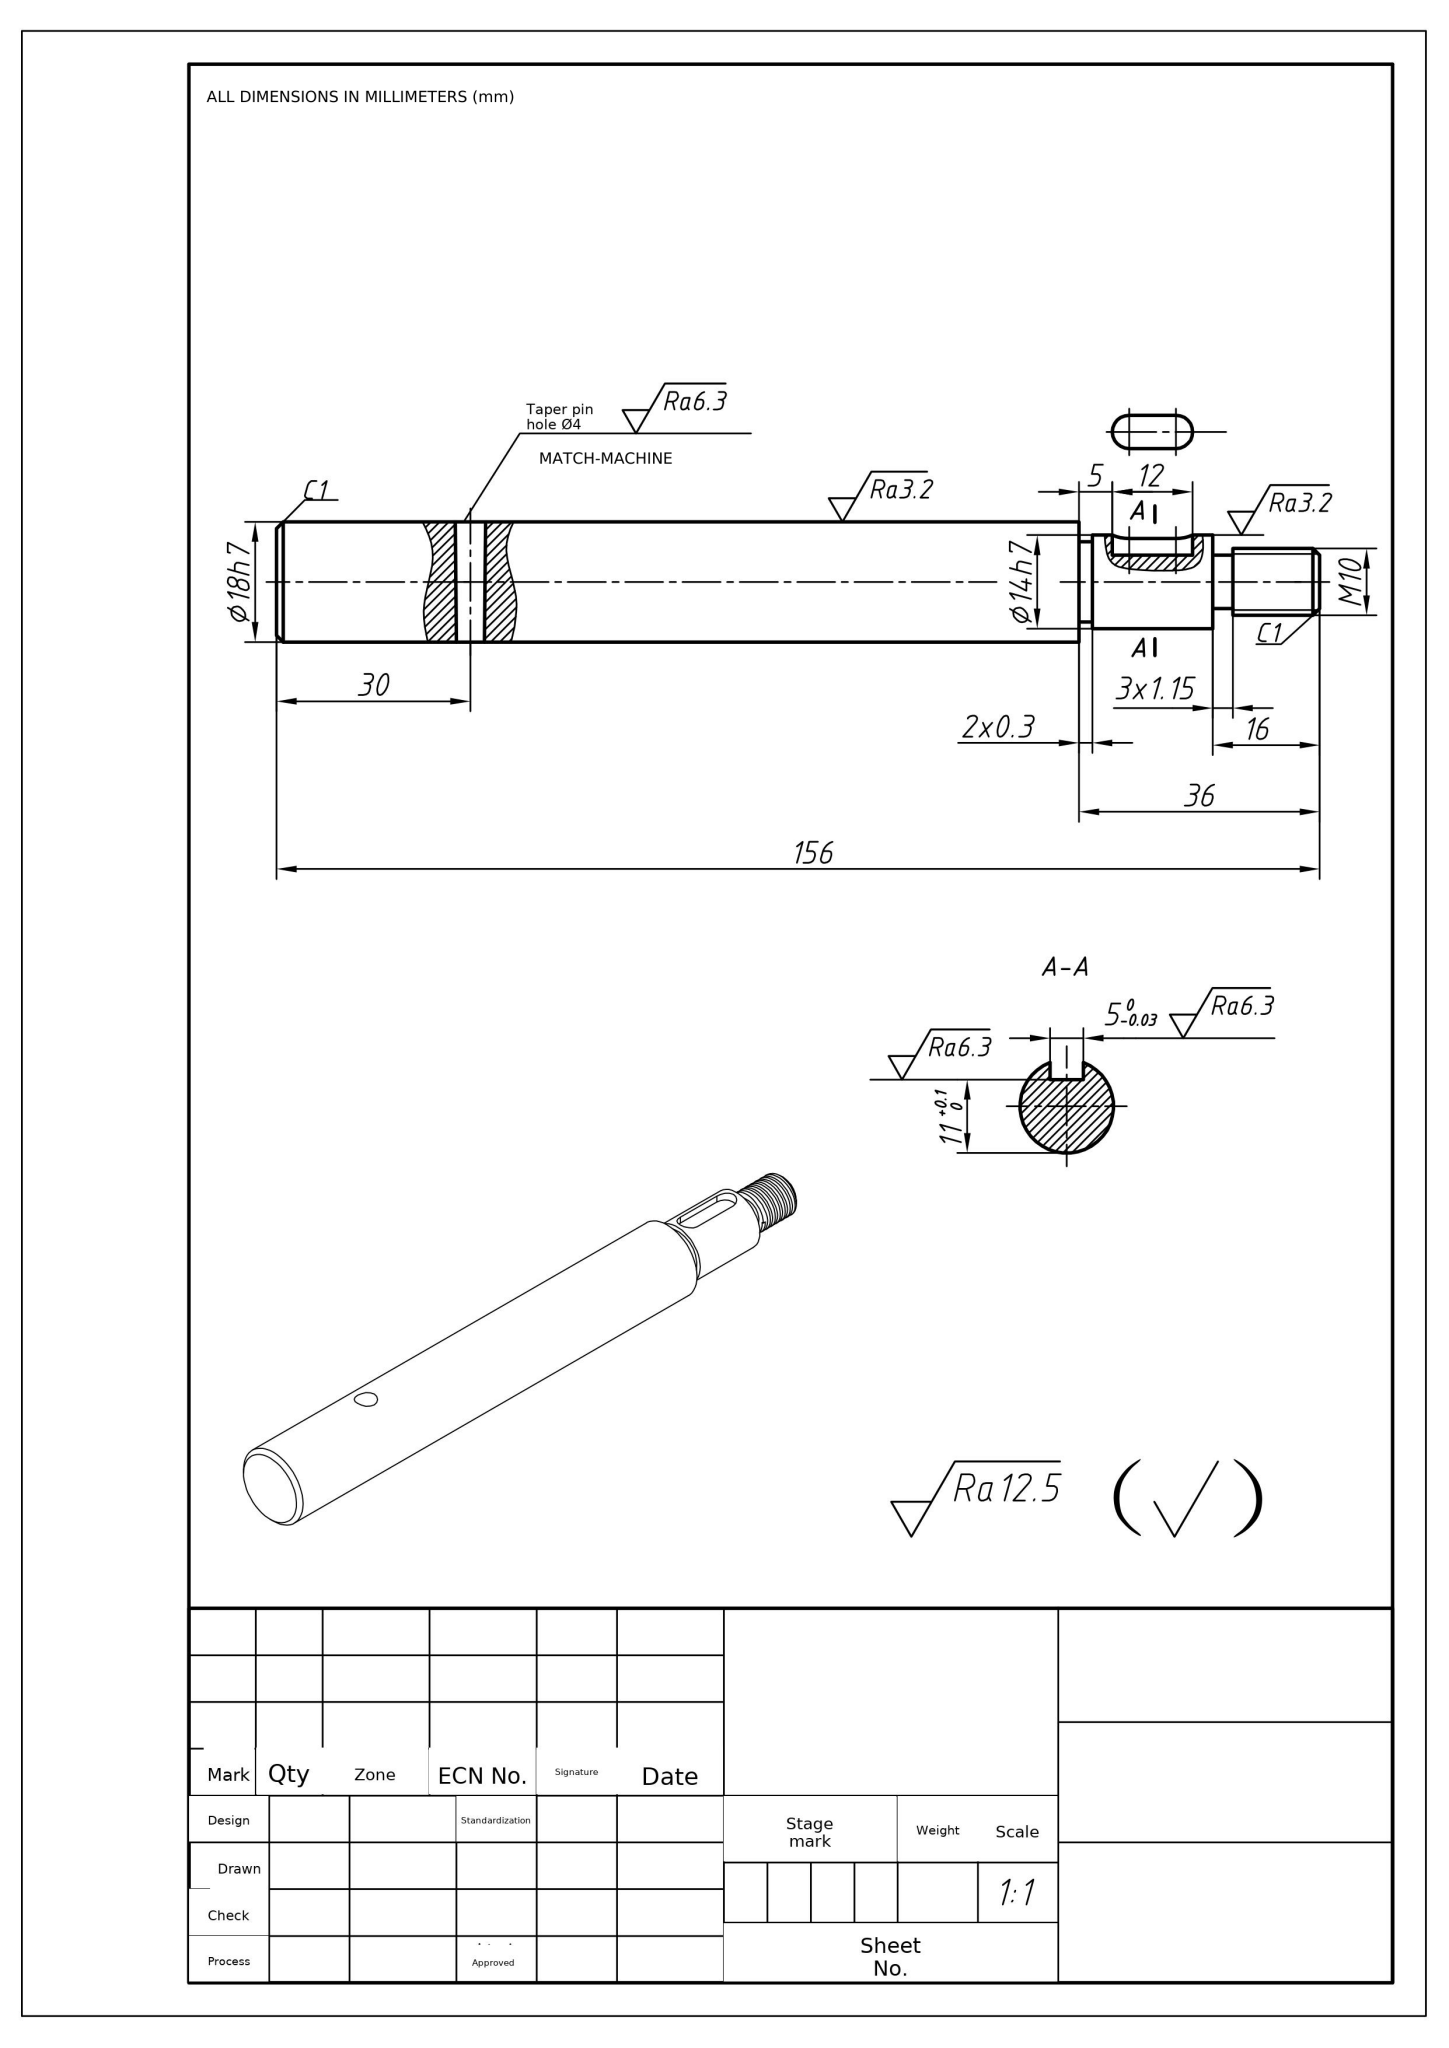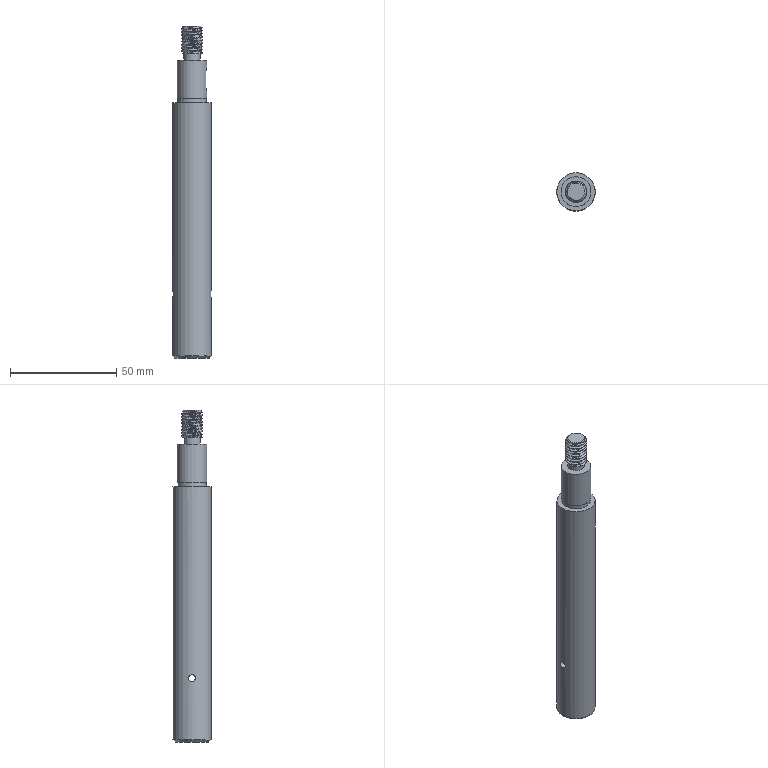Part | NX | mm | 1 solid | 23 faces | box 18 x 18 x 156 mm | volume 34216 mm3 | plane 10 | cylinder 8 | cone 3 | spline 2 | commonest cylinder face diameters 5 x2 14 x1 18 x1 13.4 x1 7.7 x1 10 x1 8.5 x1